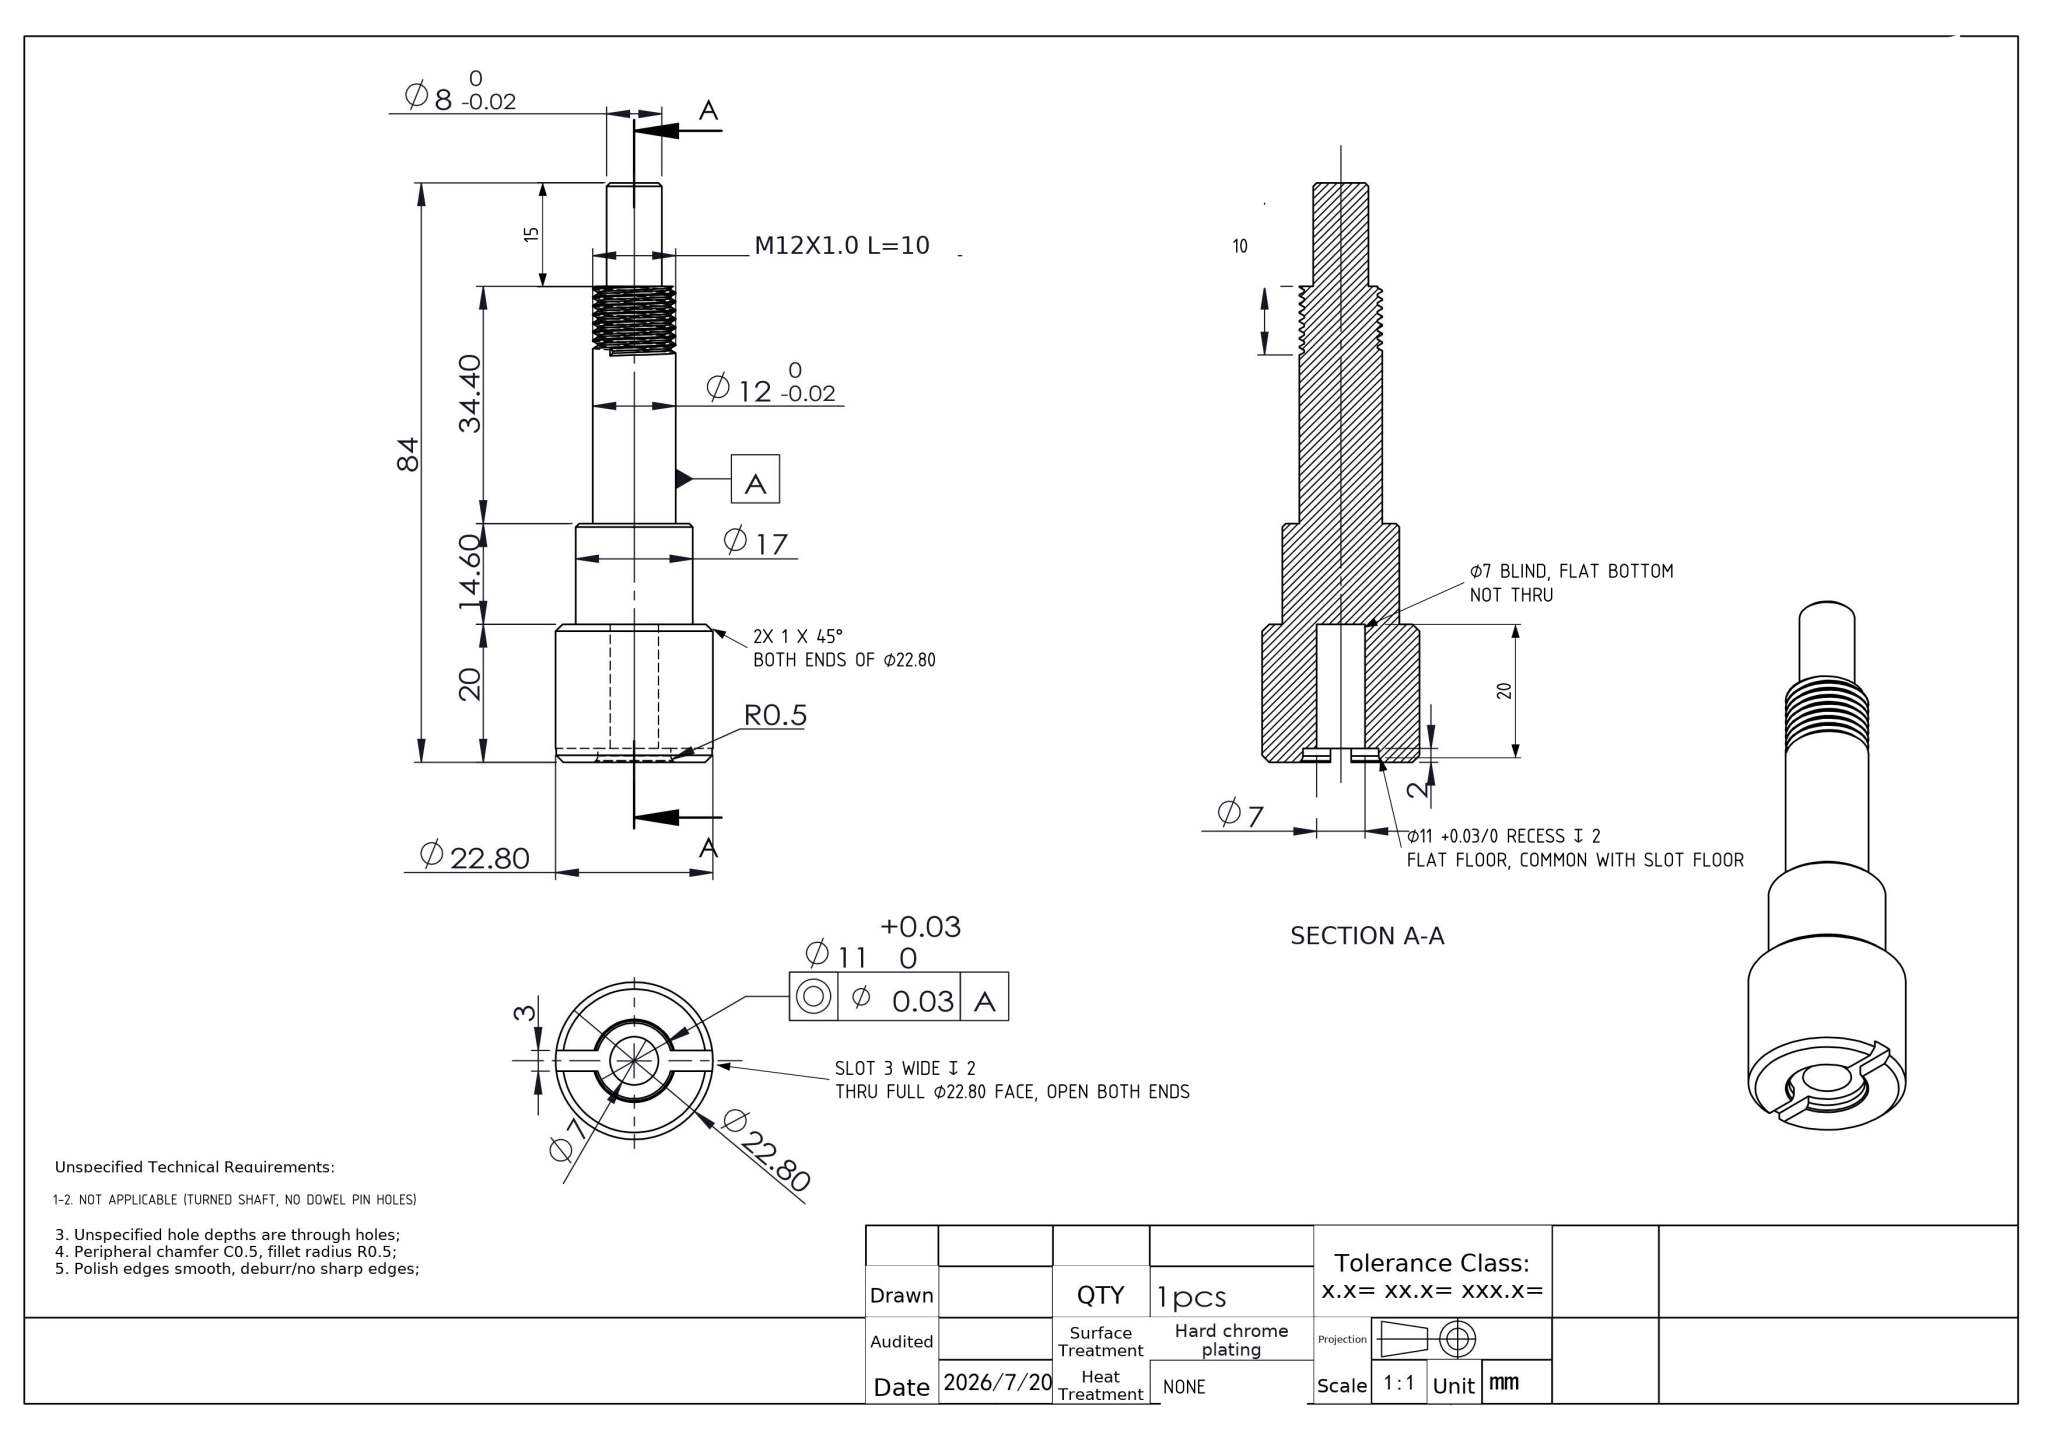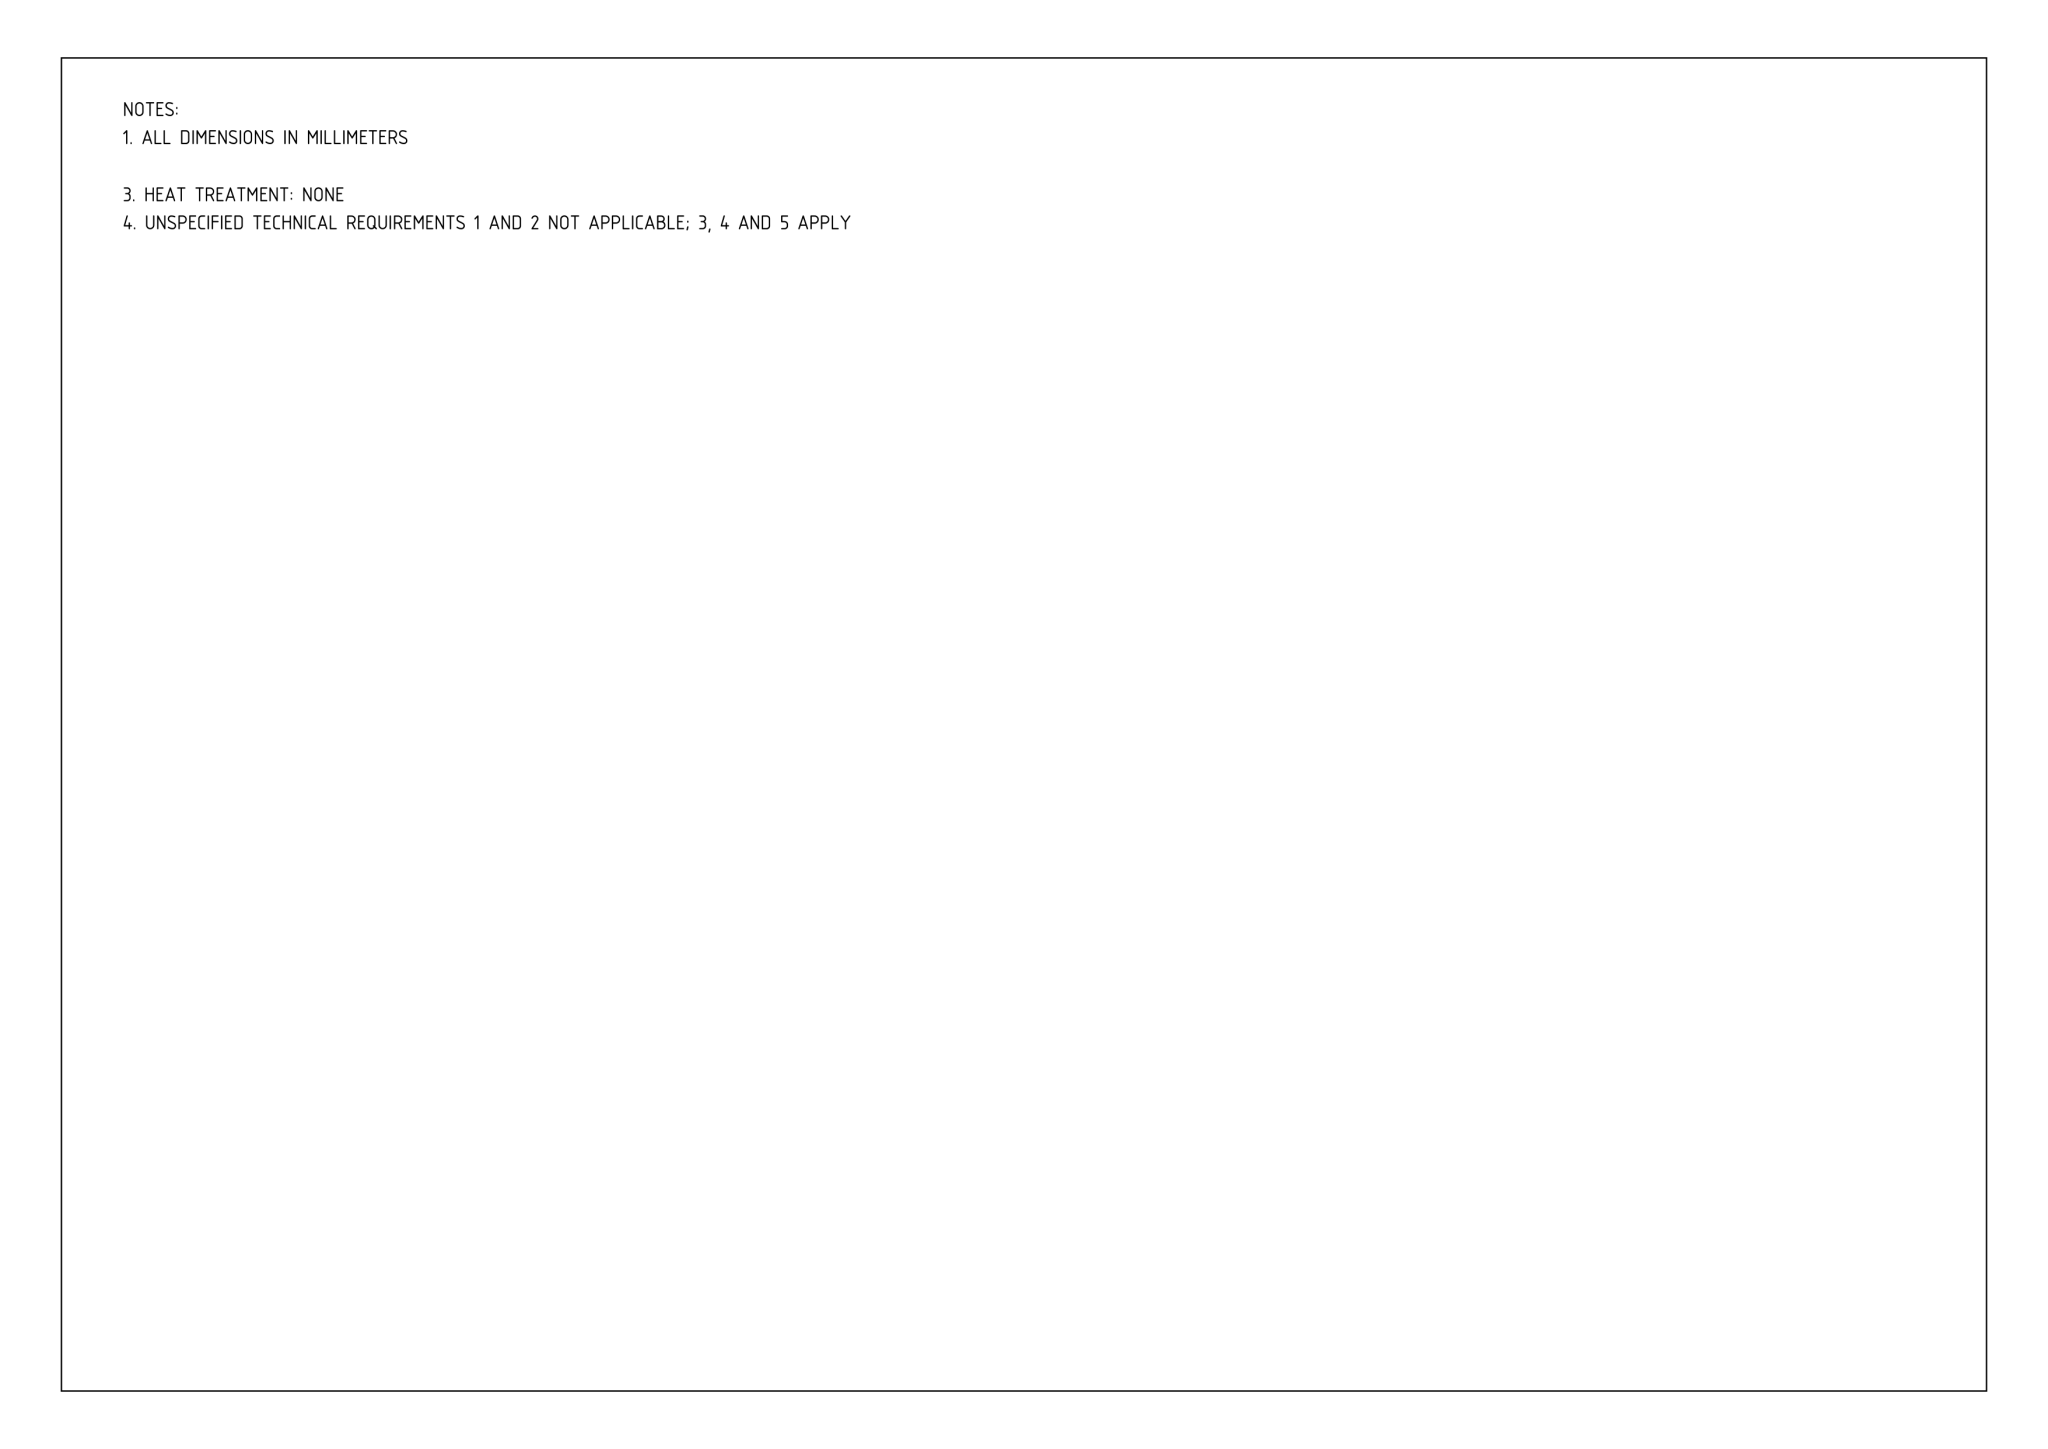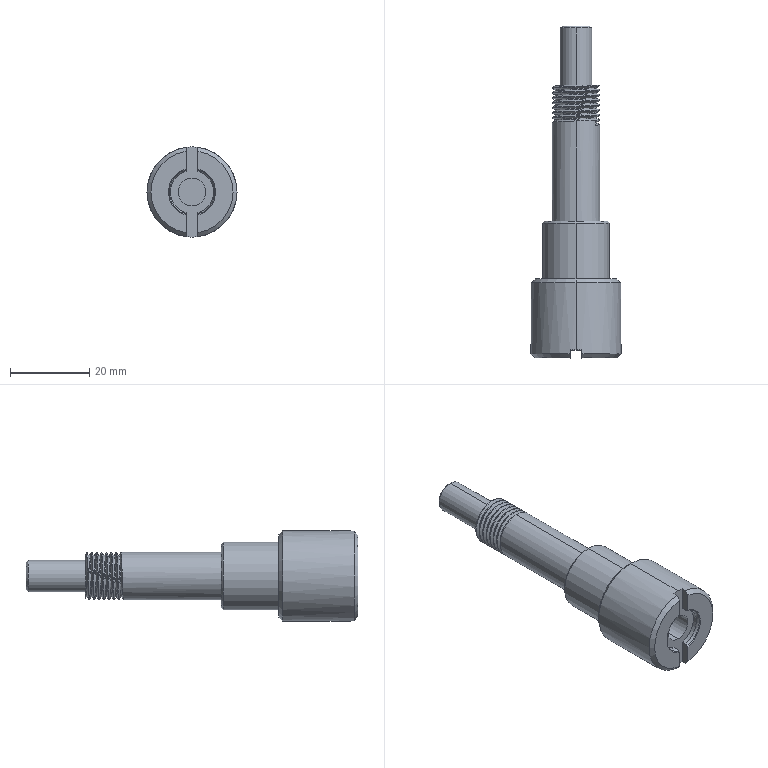Part | NX | mm | 1 solid | 54 faces | box 22.8 x 84 x 22.8 mm | volume 14958 mm3 | cylinder 26 | plane 13 | cone 10 | spline 3 | torus 2 | commonest cylinder face diameters 12 x16 7 x2 22.8 x2 17 x2 8 x2 11 x2